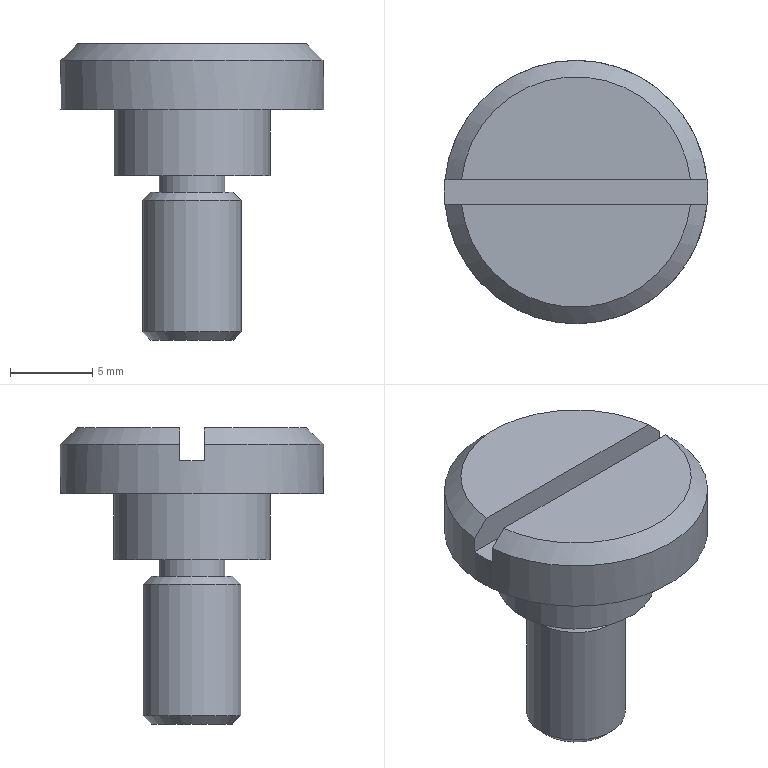Component | NX | DRILL_BUSHING_SCREW_3 | 1 solid | 17 faces | box 16 x 16 x 18 mm | volume 1280 mm3 | plane 9 | cylinder 4 | cone 4 | commonest cylinder face diameters 6 x1 4 x1 9.5 x1 16 x1
STEP:
#1=CARTESIAN_POINT('',(0.,0.,0.));
#2=DIRECTION('',(0.,0.,1.));
#3=DIRECTION('',(1.,0.,0.));
#4=AXIS2_PLACEMENT_3D('',#1,#2,#3);
#5=CARTESIAN_POINT('',(329.141,43.75,118.));
#6=VERTEX_POINT('',#5);
#7=CARTESIAN_POINT('',(343.061,43.75,118.));
#8=VERTEX_POINT('',#7);
#9=CARTESIAN_POINT('',(322.351,43.75,118.));
#10=DIRECTION('',(1.,0.,0.));
#11=VECTOR('',#10,1.);
#12=LINE('',#9,#11);
#13=CARTESIAN_POINT('',(336.101,44.5,118.));
#14=DIRECTION('',(0.,0.,1.));
#15=DIRECTION('',(1.,0.,0.));
#16=AXIS2_PLACEMENT_3D('',#13,#14,#15);
#17=PLANE('',#16);
#18=CARTESIAN_POINT('',(-13.75,-0.75));
#19=DIRECTION('',(1.,0.));
#20=VECTOR('',#19,1.);
#21=LINE('',#18,#20);
#22=(GEOMETRIC_REPRESENTATION_CONTEXT(2)PARAMETRIC_REPRESENTATION_CONTEXT()REPRESENTATION_CONTEXT('',''));
#23=DEFINITIONAL_REPRESENTATION('',(#21),#22);
#24=PCURVE('',#17,#23);
#25=CARTESIAN_POINT('',(322.351,43.75,116.));
#26=DIRECTION('',(0.,-1.,0.));
#27=DIRECTION('',(0.,0.,-1.));
#28=AXIS2_PLACEMENT_3D('',#25,#26,#27);
#29=PLANE('',#28);
#30=CARTESIAN_POINT('',(-2.,0.));
#31=DIRECTION('',(0.,1.));
#32=VECTOR('',#31,1.);
#33=LINE('',#30,#32);
#34=(GEOMETRIC_REPRESENTATION_CONTEXT(2)PARAMETRIC_REPRESENTATION_CONTEXT()REPRESENTATION_CONTEXT('',''));
#35=DEFINITIONAL_REPRESENTATION('',(#33),#34);
#36=PCURVE('',#29,#35);
#37=SURFACE_CURVE('',#12,(#24,#36),.PCURVE_S1.);
#38=EDGE_CURVE('',#6,#8,#37,.T.);
#39=ORIENTED_EDGE('',*,*,#38,.F.);
#40=CARTESIAN_POINT('',(336.101,44.5,118.));
#41=DIRECTION('',(0.,0.,1.));
#42=DIRECTION('',(1.,0.,0.));
#43=AXIS2_PLACEMENT_3D('',#40,#41,#42);
#44=CIRCLE('',#43,7.);
#45=CARTESIAN_POINT('',(0.,0.));
#46=DIRECTION('',(1.,0.));
#47=AXIS2_PLACEMENT_2D('',#45,#46);
#48=CIRCLE('',#47,7.);
#49=(GEOMETRIC_REPRESENTATION_CONTEXT(2)PARAMETRIC_REPRESENTATION_CONTEXT()REPRESENTATION_CONTEXT('',''));
#50=DEFINITIONAL_REPRESENTATION('',(#48),#49);
#51=PCURVE('',#17,#50);
#52=CARTESIAN_POINT('',(336.101,44.5,117.));
#53=DIRECTION('',(0.,0.,-1.));
#54=DIRECTION('',(-1.,0.,0.));
#55=AXIS2_PLACEMENT_3D('',#52,#53,#54);
#56=CONICAL_SURFACE('',#55,8.,0.7854);
#57=CARTESIAN_POINT('',(9.425,-1.));
#58=DIRECTION('',(-1.,-0.));
#59=VECTOR('',#58,1.);
#60=LINE('',#57,#59);
#61=(GEOMETRIC_REPRESENTATION_CONTEXT(2)PARAMETRIC_REPRESENTATION_CONTEXT()REPRESENTATION_CONTEXT('',''));
#62=DEFINITIONAL_REPRESENTATION('',(#60),#61);
#63=PCURVE('',#56,#62);
#64=SURFACE_CURVE('',#44,(#51,#63),.PCURVE_S1.);
#65=EDGE_CURVE('',#6,#8,#64,.T.);
#66=ORIENTED_EDGE('',*,*,#65,.T.);
#67=EDGE_LOOP('',(#39,#66));
#68=FACE_BOUND('',#67,.T.);
#69=ADVANCED_FACE('',(#68),#17,.T.);
#70=CARTESIAN_POINT('',(338.601,44.5,109.));
#71=VERTEX_POINT('',#70);
#72=CARTESIAN_POINT('',(336.101,44.5,109.));
#73=DIRECTION('',(0.,0.,1.));
#74=DIRECTION('',(1.,0.,0.));
#75=AXIS2_PLACEMENT_3D('',#72,#73,#74);
#76=CIRCLE('',#75,2.5);
#77=CARTESIAN_POINT('',(336.101,44.5,109.));
#78=DIRECTION('',(0.,0.,1.));
#79=DIRECTION('',(1.,0.,0.));
#80=AXIS2_PLACEMENT_3D('',#77,#78,#79);
#81=PLANE('',#80);
#82=CARTESIAN_POINT('',(0.,0.));
#83=DIRECTION('',(1.,0.));
#84=AXIS2_PLACEMENT_2D('',#82,#83);
#85=CIRCLE('',#84,2.5);
#86=(GEOMETRIC_REPRESENTATION_CONTEXT(2)PARAMETRIC_REPRESENTATION_CONTEXT()REPRESENTATION_CONTEXT('',''));
#87=DEFINITIONAL_REPRESENTATION('',(#85),#86);
#88=PCURVE('',#81,#87);
#89=CARTESIAN_POINT('',(336.101,44.5,108.5));
#90=DIRECTION('',(0.,0.,-1.));
#91=DIRECTION('',(-1.,0.,0.));
#92=AXIS2_PLACEMENT_3D('',#89,#90,#91);
#93=CONICAL_SURFACE('',#92,3.,0.7854);
#94=CARTESIAN_POINT('',(9.425,-0.5));
#95=DIRECTION('',(-1.,0.));
#96=VECTOR('',#95,1.);
#97=LINE('',#94,#96);
#98=(GEOMETRIC_REPRESENTATION_CONTEXT(2)PARAMETRIC_REPRESENTATION_CONTEXT()REPRESENTATION_CONTEXT('',''));
#99=DEFINITIONAL_REPRESENTATION('',(#97),#98);
#100=PCURVE('',#93,#99);
#101=SURFACE_CURVE('',#76,(#88,#100),.PCURVE_S1.);
#102=EDGE_CURVE('',#71,#71,#101,.T.);
#103=ORIENTED_EDGE('',*,*,#102,.T.);
#104=EDGE_LOOP('',(#103));
#105=FACE_BOUND('',#104,.T.);
#106=CARTESIAN_POINT('',(338.101,44.5,109.));
#107=VERTEX_POINT('',#106);
#108=CARTESIAN_POINT('',(336.101,44.5,109.));
#109=DIRECTION('',(0.,0.,1.));
#110=DIRECTION('',(1.,0.,0.));
#111=AXIS2_PLACEMENT_3D('',#108,#109,#110);
#112=CIRCLE('',#111,2.);
#113=CARTESIAN_POINT('',(0.,0.));
#114=DIRECTION('',(1.,0.));
#115=AXIS2_PLACEMENT_2D('',#113,#114);
#116=CIRCLE('',#115,2.);
#117=(GEOMETRIC_REPRESENTATION_CONTEXT(2)PARAMETRIC_REPRESENTATION_CONTEXT()REPRESENTATION_CONTEXT('',''));
#118=DEFINITIONAL_REPRESENTATION('',(#116),#117);
#119=PCURVE('',#81,#118);
#120=CARTESIAN_POINT('',(336.101,44.5,109.));
#121=DIRECTION('',(0.,0.,1.));
#122=DIRECTION('',(1.,0.,0.));
#123=AXIS2_PLACEMENT_3D('',#120,#121,#122);
#124=CYLINDRICAL_SURFACE('',#123,2.);
#125=CARTESIAN_POINT('',(0.,0.));
#126=DIRECTION('',(1.,0.));
#127=VECTOR('',#126,1.);
#128=LINE('',#125,#127);
#129=(GEOMETRIC_REPRESENTATION_CONTEXT(2)PARAMETRIC_REPRESENTATION_CONTEXT()REPRESENTATION_CONTEXT('',''));
#130=DEFINITIONAL_REPRESENTATION('',(#128),#129);
#131=PCURVE('',#124,#130);
#132=SURFACE_CURVE('',#112,(#119,#131),.PCURVE_S1.);
#133=EDGE_CURVE('',#107,#107,#132,.T.);
#134=ORIENTED_EDGE('',*,*,#133,.F.);
#135=EDGE_LOOP('',(#134));
#136=FACE_BOUND('',#135,.T.);
#137=ADVANCED_FACE('',(#105,#136),#81,.T.);
#138=CARTESIAN_POINT('',(333.601,44.5,100.));
#139=VERTEX_POINT('',#138);
#140=CARTESIAN_POINT('',(336.101,44.5,100.));
#141=DIRECTION('',(0.,0.,-1.));
#142=DIRECTION('',(-1.,0.,0.));
#143=AXIS2_PLACEMENT_3D('',#140,#141,#142);
#144=CIRCLE('',#143,2.5);
#145=CARTESIAN_POINT('',(336.101,44.5,100.));
#146=DIRECTION('',(0.,0.,-1.));
#147=DIRECTION('',(-1.,0.,0.));
#148=AXIS2_PLACEMENT_3D('',#145,#146,#147);
#149=PLANE('',#148);
#150=CARTESIAN_POINT('',(0.,0.));
#151=DIRECTION('',(1.,0.));
#152=AXIS2_PLACEMENT_2D('',#150,#151);
#153=CIRCLE('',#152,2.5);
#154=(GEOMETRIC_REPRESENTATION_CONTEXT(2)PARAMETRIC_REPRESENTATION_CONTEXT()REPRESENTATION_CONTEXT('',''));
#155=DEFINITIONAL_REPRESENTATION('',(#153),#154);
#156=PCURVE('',#149,#155);
#157=CARTESIAN_POINT('',(336.101,44.5,100.5));
#158=DIRECTION('',(0.,0.,1.));
#159=DIRECTION('',(1.,0.,0.));
#160=AXIS2_PLACEMENT_3D('',#157,#158,#159);
#161=CONICAL_SURFACE('',#160,3.,0.7854);
#162=CARTESIAN_POINT('',(9.425,-0.5));
#163=DIRECTION('',(-1.,0.));
#164=VECTOR('',#163,1.);
#165=LINE('',#162,#164);
#166=(GEOMETRIC_REPRESENTATION_CONTEXT(2)PARAMETRIC_REPRESENTATION_CONTEXT()REPRESENTATION_CONTEXT('',''));
#167=DEFINITIONAL_REPRESENTATION('',(#165),#166);
#168=PCURVE('',#161,#167);
#169=SURFACE_CURVE('',#144,(#156,#168),.PCURVE_S1.);
#170=EDGE_CURVE('',#139,#139,#169,.T.);
#171=ORIENTED_EDGE('',*,*,#170,.T.);
#172=EDGE_LOOP('',(#171));
#173=FACE_BOUND('',#172,.T.);
#174=ADVANCED_FACE('',(#173),#149,.T.);
#175=CARTESIAN_POINT('',(333.101,44.5,100.5));
#176=VERTEX_POINT('',#175);
#177=CARTESIAN_POINT('',(339.101,44.5,100.5));
#178=VERTEX_POINT('',#177);
#179=CARTESIAN_POINT('',(336.101,44.5,100.5));
#180=DIRECTION('',(0.,0.,1.));
#181=DIRECTION('',(-1.,0.,0.));
#182=AXIS2_PLACEMENT_3D('',#179,#180,#181);
#183=CIRCLE('',#182,3.);
#184=CARTESIAN_POINT('',(336.101,44.5,100.));
#185=DIRECTION('',(0.,0.,1.));
#186=DIRECTION('',(1.,0.,0.));
#187=AXIS2_PLACEMENT_3D('',#184,#185,#186);
#188=CYLINDRICAL_SURFACE('',#187,3.);
#189=CARTESIAN_POINT('',(3.142,0.5));
#190=DIRECTION('',(1.,0.));
#191=VECTOR('',#190,1.);
#192=LINE('',#189,#191);
#193=(GEOMETRIC_REPRESENTATION_CONTEXT(2)PARAMETRIC_REPRESENTATION_CONTEXT()REPRESENTATION_CONTEXT('',''));
#194=DEFINITIONAL_REPRESENTATION('',(#192),#193);
#195=PCURVE('',#188,#194);
#196=CARTESIAN_POINT('',(3.142,0.));
#197=DIRECTION('',(1.,0.));
#198=VECTOR('',#197,1.);
#199=LINE('',#196,#198);
#200=(GEOMETRIC_REPRESENTATION_CONTEXT(2)PARAMETRIC_REPRESENTATION_CONTEXT()REPRESENTATION_CONTEXT('',''));
#201=DEFINITIONAL_REPRESENTATION('',(#199),#200);
#202=PCURVE('',#161,#201);
#203=SURFACE_CURVE('',#183,(#195,#202),.PCURVE_S1.);
#204=EDGE_CURVE('',#176,#178,#203,.T.);
#205=ORIENTED_EDGE('',*,*,#204,.T.);
#206=CARTESIAN_POINT('',(339.101,44.5,108.5));
#207=VERTEX_POINT('',#206);
#208=CARTESIAN_POINT('',(339.101,44.5,100.5));
#209=CARTESIAN_POINT('',(339.101,44.5,108.5));
#210=B_SPLINE_CURVE_WITH_KNOTS('',1,(#208,#209),.UNSPECIFIED.,.F.,.F.,(2,2),(0.5,8.5),.PIECEWISE_BEZIER_KNOTS.);
#211=CARTESIAN_POINT('',(6.283,0.));
#212=DIRECTION('',(0.,1.));
#213=VECTOR('',#212,1.);
#214=LINE('',#211,#213);
#215=(GEOMETRIC_REPRESENTATION_CONTEXT(2)PARAMETRIC_REPRESENTATION_CONTEXT()REPRESENTATION_CONTEXT('',''));
#216=DEFINITIONAL_REPRESENTATION('',(#214),#215);
#217=PCURVE('',#188,#216);
#218=CARTESIAN_POINT('',(0.,0.));
#219=DIRECTION('',(0.,1.));
#220=VECTOR('',#219,1.);
#221=LINE('',#218,#220);
#222=(GEOMETRIC_REPRESENTATION_CONTEXT(2)PARAMETRIC_REPRESENTATION_CONTEXT()REPRESENTATION_CONTEXT('',''));
#223=DEFINITIONAL_REPRESENTATION('',(#221),#222);
#224=PCURVE('',#188,#223);
#225=SEAM_CURVE('',#210,(#217,#224),.PCURVE_S1.);
#226=EDGE_CURVE('',#178,#207,#225,.T.);
#227=ORIENTED_EDGE('',*,*,#226,.T.);
#228=CARTESIAN_POINT('',(336.101,44.5,108.5));
#229=DIRECTION('',(0.,0.,-1.));
#230=DIRECTION('',(1.,0.,0.));
#231=AXIS2_PLACEMENT_3D('',#228,#229,#230);
#232=CIRCLE('',#231,3.);
#233=CARTESIAN_POINT('',(6.283,8.5));
#234=DIRECTION('',(-1.,0.));
#235=VECTOR('',#234,1.);
#236=LINE('',#233,#235);
#237=(GEOMETRIC_REPRESENTATION_CONTEXT(2)PARAMETRIC_REPRESENTATION_CONTEXT()REPRESENTATION_CONTEXT('',''));
#238=DEFINITIONAL_REPRESENTATION('',(#236),#237);
#239=PCURVE('',#188,#238);
#240=CARTESIAN_POINT('',(3.142,0.));
#241=DIRECTION('',(1.,0.));
#242=VECTOR('',#241,1.);
#243=LINE('',#240,#242);
#244=(GEOMETRIC_REPRESENTATION_CONTEXT(2)PARAMETRIC_REPRESENTATION_CONTEXT()REPRESENTATION_CONTEXT('',''));
#245=DEFINITIONAL_REPRESENTATION('',(#243),#244);
#246=PCURVE('',#93,#245);
#247=SURFACE_CURVE('',#232,(#239,#246),.PCURVE_S1.);
#248=EDGE_CURVE('',#207,#207,#247,.T.);
#249=ORIENTED_EDGE('',*,*,#248,.T.);
#250=ORIENTED_EDGE('',*,*,#226,.F.);
#251=CARTESIAN_POINT('',(336.101,44.5,100.5));
#252=DIRECTION('',(0.,0.,1.));
#253=DIRECTION('',(-1.,0.,0.));
#254=AXIS2_PLACEMENT_3D('',#251,#252,#253);
#255=CIRCLE('',#254,3.);
#256=CARTESIAN_POINT('',(-3.142,0.5));
#257=DIRECTION('',(1.,0.));
#258=VECTOR('',#257,1.);
#259=LINE('',#256,#258);
#260=(GEOMETRIC_REPRESENTATION_CONTEXT(2)PARAMETRIC_REPRESENTATION_CONTEXT()REPRESENTATION_CONTEXT('',''));
#261=DEFINITIONAL_REPRESENTATION('',(#259),#260);
#262=PCURVE('',#188,#261);
#263=CARTESIAN_POINT('',(3.142,0.));
#264=DIRECTION('',(1.,0.));
#265=VECTOR('',#264,1.);
#266=LINE('',#263,#265);
#267=(GEOMETRIC_REPRESENTATION_CONTEXT(2)PARAMETRIC_REPRESENTATION_CONTEXT()REPRESENTATION_CONTEXT('',''));
#268=DEFINITIONAL_REPRESENTATION('',(#266),#267);
#269=PCURVE('',#161,#268);
#270=SURFACE_CURVE('',#255,(#262,#269),.PCURVE_S1.);
#271=EDGE_CURVE('',#178,#176,#270,.T.);
#272=ORIENTED_EDGE('',*,*,#271,.T.);
#273=EDGE_LOOP('',(#205,#227,#249,#250,#272));
#274=FACE_BOUND('',#273,.T.);
#275=ADVANCED_FACE('',(#274),#188,.T.);
#276=CARTESIAN_POINT('',(338.101,44.5,110.));
#277=VERTEX_POINT('',#276);
#278=CARTESIAN_POINT('',(336.101,44.5,110.));
#279=DIRECTION('',(0.,0.,-1.));
#280=DIRECTION('',(1.,0.,0.));
#281=AXIS2_PLACEMENT_3D('',#278,#279,#280);
#282=CIRCLE('',#281,2.);
#283=CARTESIAN_POINT('',(6.283,1.));
#284=DIRECTION('',(-1.,0.));
#285=VECTOR('',#284,1.);
#286=LINE('',#283,#285);
#287=(GEOMETRIC_REPRESENTATION_CONTEXT(2)PARAMETRIC_REPRESENTATION_CONTEXT()REPRESENTATION_CONTEXT('',''));
#288=DEFINITIONAL_REPRESENTATION('',(#286),#287);
#289=PCURVE('',#124,#288);
#290=CARTESIAN_POINT('',(336.101,44.5,110.));
#291=DIRECTION('',(0.,0.,-1.));
#292=DIRECTION('',(-1.,0.,0.));
#293=AXIS2_PLACEMENT_3D('',#290,#291,#292);
#294=PLANE('',#293);
#295=CARTESIAN_POINT('',(0.,0.));
#296=DIRECTION('',(-1.,0.));
#297=AXIS2_PLACEMENT_2D('',#295,#296);
#298=CIRCLE('',#297,2.);
#299=(GEOMETRIC_REPRESENTATION_CONTEXT(2)PARAMETRIC_REPRESENTATION_CONTEXT()REPRESENTATION_CONTEXT('',''));
#300=DEFINITIONAL_REPRESENTATION('',(#298),#299);
#301=PCURVE('',#294,#300);
#302=SURFACE_CURVE('',#282,(#289,#301),.PCURVE_S1.);
#303=EDGE_CURVE('',#277,#277,#302,.T.);
#304=ORIENTED_EDGE('',*,*,#303,.T.);
#305=CARTESIAN_POINT('',(338.101,44.5,109.));
#306=CARTESIAN_POINT('',(338.101,44.5,110.));
#307=B_SPLINE_CURVE_WITH_KNOTS('',1,(#305,#306),.UNSPECIFIED.,.F.,.F.,(2,2),(0.,1.),.PIECEWISE_BEZIER_KNOTS.);
#308=CARTESIAN_POINT('',(0.,0.));
#309=DIRECTION('',(0.,1.));
#310=VECTOR('',#309,1.);
#311=LINE('',#308,#310);
#312=(GEOMETRIC_REPRESENTATION_CONTEXT(2)PARAMETRIC_REPRESENTATION_CONTEXT()REPRESENTATION_CONTEXT('',''));
#313=DEFINITIONAL_REPRESENTATION('',(#311),#312);
#314=PCURVE('',#124,#313);
#315=CARTESIAN_POINT('',(6.283,0.));
#316=DIRECTION('',(0.,1.));
#317=VECTOR('',#316,1.);
#318=LINE('',#315,#317);
#319=(GEOMETRIC_REPRESENTATION_CONTEXT(2)PARAMETRIC_REPRESENTATION_CONTEXT()REPRESENTATION_CONTEXT('',''));
#320=DEFINITIONAL_REPRESENTATION('',(#318),#319);
#321=PCURVE('',#124,#320);
#322=SEAM_CURVE('',#307,(#314,#321),.PCURVE_S1.);
#323=EDGE_CURVE('',#107,#277,#322,.T.);
#324=ORIENTED_EDGE('',*,*,#323,.F.);
#325=ORIENTED_EDGE('',*,*,#133,.T.);
#326=ORIENTED_EDGE('',*,*,#323,.T.);
#327=EDGE_LOOP('',(#304,#324,#325,#326));
#328=FACE_BOUND('',#327,.T.);
#329=ADVANCED_FACE('',(#328),#124,.T.);
#330=ORIENTED_EDGE('',*,*,#303,.F.);
#331=EDGE_LOOP('',(#330));
#332=FACE_BOUND('',#331,.T.);
#333=CARTESIAN_POINT('',(340.851,44.5,110.));
#334=VERTEX_POINT('',#333);
#335=CARTESIAN_POINT('',(336.101,44.5,110.));
#336=DIRECTION('',(0.,0.,1.));
#337=DIRECTION('',(1.,0.,0.));
#338=AXIS2_PLACEMENT_3D('',#335,#336,#337);
#339=CIRCLE('',#338,4.75);
#340=CARTESIAN_POINT('',(-4.75,0.));
#341=CARTESIAN_POINT('',(-4.75,8.227));
#342=CARTESIAN_POINT('',(2.375,4.114));
#343=CARTESIAN_POINT('',(9.5,0.));
#344=CARTESIAN_POINT('',(2.375,-4.114));
#345=CARTESIAN_POINT('',(-4.75,-8.227));
#346=CARTESIAN_POINT('',(-4.75,0.));
#347=(BOUNDED_CURVE()B_SPLINE_CURVE(2,(#340,#341,#342,#343,#344,#345,#346),.UNSPECIFIED.,.T.,.F.)B_SPLINE_CURVE_WITH_KNOTS((1,2,2,2,2,1),(-2.094,0.,2.094,4.189,6.283,8.378),.UNSPECIFIED.)CURVE()GEOMETRIC_REPRESENTATION_ITEM()RATIONAL_B_SPLINE_CURVE((1.,0.5,1.,0.5,1.,0.5,1.))REPRESENTATION_ITEM(''));
#348=(GEOMETRIC_REPRESENTATION_CONTEXT(2)PARAMETRIC_REPRESENTATION_CONTEXT()REPRESENTATION_CONTEXT('',''));
#349=DEFINITIONAL_REPRESENTATION('',(#347),#348);
#350=PCURVE('',#294,#349);
#351=CARTESIAN_POINT('',(336.101,44.5,110.));
#352=DIRECTION('',(0.,0.,1.));
#353=DIRECTION('',(1.,0.,0.));
#354=AXIS2_PLACEMENT_3D('',#351,#352,#353);
#355=CYLINDRICAL_SURFACE('',#354,4.75);
#356=CARTESIAN_POINT('',(0.,0.));
#357=DIRECTION('',(1.,0.));
#358=VECTOR('',#357,1.);
#359=LINE('',#356,#358);
#360=(GEOMETRIC_REPRESENTATION_CONTEXT(2)PARAMETRIC_REPRESENTATION_CONTEXT()REPRESENTATION_CONTEXT('',''));
#361=DEFINITIONAL_REPRESENTATION('',(#359),#360);
#362=PCURVE('',#355,#361);
#363=SURFACE_CURVE('',#339,(#350,#362),.PCURVE_S1.);
#364=EDGE_CURVE('',#334,#334,#363,.T.);
#365=ORIENTED_EDGE('',*,*,#364,.F.);
#366=EDGE_LOOP('',(#365));
#367=FACE_BOUND('',#366,.T.);
#368=ADVANCED_FACE('',(#332,#367),#294,.T.);
#369=CARTESIAN_POINT('',(340.851,44.5,114.));
#370=VERTEX_POINT('',#369);
#371=CARTESIAN_POINT('',(336.101,44.5,114.));
#372=DIRECTION('',(0.,0.,-1.));
#373=DIRECTION('',(1.,0.,0.));
#374=AXIS2_PLACEMENT_3D('',#371,#372,#373);
#375=CIRCLE('',#374,4.75);
#376=CARTESIAN_POINT('',(6.283,4.));
#377=DIRECTION('',(-1.,0.));
#378=VECTOR('',#377,1.);
#379=LINE('',#376,#378);
#380=(GEOMETRIC_REPRESENTATION_CONTEXT(2)PARAMETRIC_REPRESENTATION_CONTEXT()REPRESENTATION_CONTEXT('',''));
#381=DEFINITIONAL_REPRESENTATION('',(#379),#380);
#382=PCURVE('',#355,#381);
#383=CARTESIAN_POINT('',(336.101,44.5,114.));
#384=DIRECTION('',(0.,0.,-1.));
#385=DIRECTION('',(-1.,0.,0.));
#386=AXIS2_PLACEMENT_3D('',#383,#384,#385);
#387=PLANE('',#386);
#388=CARTESIAN_POINT('',(0.,0.));
#389=DIRECTION('',(-1.,0.));
#390=AXIS2_PLACEMENT_2D('',#388,#389);
#391=CIRCLE('',#390,4.75);
#392=(GEOMETRIC_REPRESENTATION_CONTEXT(2)PARAMETRIC_REPRESENTATION_CONTEXT()REPRESENTATION_CONTEXT('',''));
#393=DEFINITIONAL_REPRESENTATION('',(#391),#392);
#394=PCURVE('',#387,#393);
#395=SURFACE_CURVE('',#375,(#382,#394),.PCURVE_S1.);
#396=EDGE_CURVE('',#370,#370,#395,.T.);
#397=ORIENTED_EDGE('',*,*,#396,.T.);
#398=CARTESIAN_POINT('',(340.851,44.5,110.));
#399=CARTESIAN_POINT('',(340.851,44.5,114.));
#400=B_SPLINE_CURVE_WITH_KNOTS('',1,(#398,#399),.UNSPECIFIED.,.F.,.F.,(2,2),(0.,4.),.PIECEWISE_BEZIER_KNOTS.);
#401=CARTESIAN_POINT('',(0.,0.));
#402=DIRECTION('',(0.,1.));
#403=VECTOR('',#402,1.);
#404=LINE('',#401,#403);
#405=(GEOMETRIC_REPRESENTATION_CONTEXT(2)PARAMETRIC_REPRESENTATION_CONTEXT()REPRESENTATION_CONTEXT('',''));
#406=DEFINITIONAL_REPRESENTATION('',(#404),#405);
#407=PCURVE('',#355,#406);
#408=CARTESIAN_POINT('',(6.283,0.));
#409=DIRECTION('',(0.,1.));
#410=VECTOR('',#409,1.);
#411=LINE('',#408,#410);
#412=(GEOMETRIC_REPRESENTATION_CONTEXT(2)PARAMETRIC_REPRESENTATION_CONTEXT()REPRESENTATION_CONTEXT('',''));
#413=DEFINITIONAL_REPRESENTATION('',(#411),#412);
#414=PCURVE('',#355,#413);
#415=SEAM_CURVE('',#400,(#407,#414),.PCURVE_S1.);
#416=EDGE_CURVE('',#334,#370,#415,.T.);
#417=ORIENTED_EDGE('',*,*,#416,.F.);
#418=ORIENTED_EDGE('',*,*,#364,.T.);
#419=ORIENTED_EDGE('',*,*,#416,.T.);
#420=EDGE_LOOP('',(#397,#417,#418,#419));
#421=FACE_BOUND('',#420,.T.);
#422=ADVANCED_FACE('',(#421),#355,.T.);
#423=CARTESIAN_POINT('',(343.061,45.25,118.));
#424=VERTEX_POINT('',#423);
#425=CARTESIAN_POINT('',(329.141,45.25,118.));
#426=VERTEX_POINT('',#425);
#427=CARTESIAN_POINT('',(349.851,45.25,118.));
#428=DIRECTION('',(-1.,0.,0.));
#429=VECTOR('',#428,1.);
#430=LINE('',#427,#429);
#431=CARTESIAN_POINT('',(336.101,44.5,118.));
#432=DIRECTION('',(0.,0.,1.));
#433=DIRECTION('',(1.,0.,0.));
#434=AXIS2_PLACEMENT_3D('',#431,#432,#433);
#435=PLANE('',#434);
#436=CARTESIAN_POINT('',(13.75,0.75));
#437=DIRECTION('',(-1.,0.));
#438=VECTOR('',#437,1.);
#439=LINE('',#436,#438);
#440=(GEOMETRIC_REPRESENTATION_CONTEXT(2)PARAMETRIC_REPRESENTATION_CONTEXT()REPRESENTATION_CONTEXT('',''));
#441=DEFINITIONAL_REPRESENTATION('',(#439),#440);
#442=PCURVE('',#435,#441);
#443=CARTESIAN_POINT('',(349.851,45.25,116.));
#444=DIRECTION('',(0.,1.,0.));
#445=DIRECTION('',(0.,0.,1.));
#446=AXIS2_PLACEMENT_3D('',#443,#444,#445);
#447=PLANE('',#446);
#448=CARTESIAN_POINT('',(2.,0.));
#449=DIRECTION('',(0.,-1.));
#450=VECTOR('',#449,1.);
#451=LINE('',#448,#450);
#452=(GEOMETRIC_REPRESENTATION_CONTEXT(2)PARAMETRIC_REPRESENTATION_CONTEXT()REPRESENTATION_CONTEXT('',''));
#453=DEFINITIONAL_REPRESENTATION('',(#451),#452);
#454=PCURVE('',#447,#453);
#455=SURFACE_CURVE('',#430,(#442,#454),.PCURVE_S1.);
#456=EDGE_CURVE('',#424,#426,#455,.T.);
#457=ORIENTED_EDGE('',*,*,#456,.F.);
#458=CARTESIAN_POINT('',(336.101,44.5,118.));
#459=DIRECTION('',(0.,0.,1.));
#460=DIRECTION('',(1.,0.,0.));
#461=AXIS2_PLACEMENT_3D('',#458,#459,#460);
#462=CIRCLE('',#461,7.);
#463=CARTESIAN_POINT('',(0.,0.));
#464=DIRECTION('',(1.,0.));
#465=AXIS2_PLACEMENT_2D('',#463,#464);
#466=CIRCLE('',#465,7.);
#467=(GEOMETRIC_REPRESENTATION_CONTEXT(2)PARAMETRIC_REPRESENTATION_CONTEXT()REPRESENTATION_CONTEXT('',''));
#468=DEFINITIONAL_REPRESENTATION('',(#466),#467);
#469=PCURVE('',#435,#468);
#470=CARTESIAN_POINT('',(336.101,44.5,117.));
#471=DIRECTION('',(0.,0.,-1.));
#472=DIRECTION('',(-1.,0.,0.));
#473=AXIS2_PLACEMENT_3D('',#470,#471,#472);
#474=CONICAL_SURFACE('',#473,8.,0.7854);
#475=CARTESIAN_POINT('',(3.142,-1.));
#476=DIRECTION('',(-1.,0.));
#477=VECTOR('',#476,1.);
#478=LINE('',#475,#477);
#479=(GEOMETRIC_REPRESENTATION_CONTEXT(2)PARAMETRIC_REPRESENTATION_CONTEXT()REPRESENTATION_CONTEXT('',''));
#480=DEFINITIONAL_REPRESENTATION('',(#478),#479);
#481=PCURVE('',#474,#480);
#482=SURFACE_CURVE('',#462,(#469,#481),.PCURVE_S1.);
#483=EDGE_CURVE('',#424,#426,#482,.T.);
#484=ORIENTED_EDGE('',*,*,#483,.T.);
#485=EDGE_LOOP('',(#457,#484));
#486=FACE_BOUND('',#485,.T.);
#487=ADVANCED_FACE('',(#486),#435,.T.);
#488=ORIENTED_EDGE('',*,*,#396,.F.);
#489=EDGE_LOOP('',(#488));
#490=FACE_BOUND('',#489,.T.);
#491=CARTESIAN_POINT('',(344.101,44.5,114.));
#492=VERTEX_POINT('',#491);
#493=CARTESIAN_POINT('',(336.101,44.5,114.));
#494=DIRECTION('',(0.,0.,1.));
#495=DIRECTION('',(1.,0.,0.));
#496=AXIS2_PLACEMENT_3D('',#493,#494,#495);
#497=CIRCLE('',#496,8.);
#498=CARTESIAN_POINT('',(-8.,0.));
#499=CARTESIAN_POINT('',(-8.,13.856));
#500=CARTESIAN_POINT('',(4.,6.928));
#501=CARTESIAN_POINT('',(16.,0.));
#502=CARTESIAN_POINT('',(4.,-6.928));
#503=CARTESIAN_POINT('',(-8.,-13.856));
#504=CARTESIAN_POINT('',(-8.,0.));
#505=(BOUNDED_CURVE()B_SPLINE_CURVE(2,(#498,#499,#500,#501,#502,#503,#504),.UNSPECIFIED.,.T.,.F.)B_SPLINE_CURVE_WITH_KNOTS((1,2,2,2,2,1),(-2.094,0.,2.094,4.189,6.283,8.378),.UNSPECIFIED.)CURVE()GEOMETRIC_REPRESENTATION_ITEM()RATIONAL_B_SPLINE_CURVE((1.,0.5,1.,0.5,1.,0.5,1.))REPRESENTATION_ITEM(''));
#506=(GEOMETRIC_REPRESENTATION_CONTEXT(2)PARAMETRIC_REPRESENTATION_CONTEXT()REPRESENTATION_CONTEXT('',''));
#507=DEFINITIONAL_REPRESENTATION('',(#505),#506);
#508=PCURVE('',#387,#507);
#509=CARTESIAN_POINT('',(336.101,44.5,114.));
#510=DIRECTION('',(0.,0.,1.));
#511=DIRECTION('',(1.,0.,0.));
#512=AXIS2_PLACEMENT_3D('',#509,#510,#511);
#513=CYLINDRICAL_SURFACE('',#512,8.);
#514=CARTESIAN_POINT('',(0.,0.));
#515=DIRECTION('',(1.,0.));
#516=VECTOR('',#515,1.);
#517=LINE('',#514,#516);
#518=(GEOMETRIC_REPRESENTATION_CONTEXT(2)PARAMETRIC_REPRESENTATION_CONTEXT()REPRESENTATION_CONTEXT('',''));
#519=DEFINITIONAL_REPRESENTATION('',(#517),#518);
#520=PCURVE('',#513,#519);
#521=SURFACE_CURVE('',#497,(#508,#520),.PCURVE_S1.);
#522=EDGE_CURVE('',#492,#492,#521,.T.);
#523=ORIENTED_EDGE('',*,*,#522,.F.);
#524=EDGE_LOOP('',(#523));
#525=FACE_BOUND('',#524,.T.);
#526=ADVANCED_FACE('',(#490,#525),#387,.T.);
#527=CARTESIAN_POINT('',(328.136,45.25,117.));
#528=VERTEX_POINT('',#527);
#529=CARTESIAN_POINT('',(328.136,45.25,116.));
#530=VERTEX_POINT('',#529);
#531=CARTESIAN_POINT('',(328.136,45.25,114.));
#532=DIRECTION('',(0.,0.,-1.));
#533=VECTOR('',#532,1.);
#534=LINE('',#531,#533);
#535=CARTESIAN_POINT('',(3.048,0.));
#536=DIRECTION('',(0.,-1.));
#537=VECTOR('',#536,1.);
#538=LINE('',#535,#537);
#539=(GEOMETRIC_REPRESENTATION_CONTEXT(2)PARAMETRIC_REPRESENTATION_CONTEXT()REPRESENTATION_CONTEXT('',''));
#540=DEFINITIONAL_REPRESENTATION('',(#538),#539);
#541=PCURVE('',#513,#540);
#542=CARTESIAN_POINT('',(-2.,-21.715));
#543=DIRECTION('',(-1.,0.));
#544=VECTOR('',#543,1.);
#545=LINE('',#542,#544);
#546=(GEOMETRIC_REPRESENTATION_CONTEXT(2)PARAMETRIC_REPRESENTATION_CONTEXT()REPRESENTATION_CONTEXT('',''));
#547=DEFINITIONAL_REPRESENTATION('',(#545),#546);
#548=PCURVE('',#447,#547);
#549=SURFACE_CURVE('',#534,(#541,#548),.PCURVE_S1.);
#550=EDGE_CURVE('',#528,#530,#549,.T.);
#551=ORIENTED_EDGE('',*,*,#550,.F.);
#552=CARTESIAN_POINT('',(344.066,45.25,117.));
#553=VERTEX_POINT('',#552);
#554=CARTESIAN_POINT('',(336.101,44.5,117.));
#555=DIRECTION('',(0.,0.,-1.));
#556=DIRECTION('',(1.,0.,0.));
#557=AXIS2_PLACEMENT_3D('',#554,#555,#556);
#558=CIRCLE('',#557,8.);
#559=CARTESIAN_POINT('',(6.283,3.));
#560=DIRECTION('',(-1.,0.));
#561=VECTOR('',#560,1.);
#562=LINE('',#559,#561);
#563=(GEOMETRIC_REPRESENTATION_CONTEXT(2)PARAMETRIC_REPRESENTATION_CONTEXT()REPRESENTATION_CONTEXT('',''));
#564=DEFINITIONAL_REPRESENTATION('',(#562),#563);
#565=PCURVE('',#513,#564);
#566=CARTESIAN_POINT('',(-3.142,0.));
#567=DIRECTION('',(1.,0.));
#568=VECTOR('',#567,1.);
#569=LINE('',#566,#568);
#570=(GEOMETRIC_REPRESENTATION_CONTEXT(2)PARAMETRIC_REPRESENTATION_CONTEXT()REPRESENTATION_CONTEXT('',''));
#571=DEFINITIONAL_REPRESENTATION('',(#569),#570);
#572=PCURVE('',#474,#571);
#573=SURFACE_CURVE('',#558,(#565,#572),.PCURVE_S1.);
#574=EDGE_CURVE('',#528,#553,#573,.T.);
#575=ORIENTED_EDGE('',*,*,#574,.T.);
#576=CARTESIAN_POINT('',(344.066,45.25,116.));
#577=VERTEX_POINT('',#576);
#578=CARTESIAN_POINT('',(344.066,45.25,114.));
#579=DIRECTION('',(0.,0.,1.));
#580=VECTOR('',#579,1.);
#581=LINE('',#578,#580);
#582=CARTESIAN_POINT('',(0.09389,0.));
#583=DIRECTION('',(0.,1.));
#584=VECTOR('',#583,1.);
#585=LINE('',#582,#584);
#586=(GEOMETRIC_REPRESENTATION_CONTEXT(2)PARAMETRIC_REPRESENTATION_CONTEXT()REPRESENTATION_CONTEXT('',''));
#587=DEFINITIONAL_REPRESENTATION('',(#585),#586);
#588=PCURVE('',#513,#587);
#589=CARTESIAN_POINT('',(-2.,-5.785));
#590=DIRECTION('',(1.,0.));
#591=VECTOR('',#590,1.);
#592=LINE('',#589,#591);
#593=(GEOMETRIC_REPRESENTATION_CONTEXT(2)PARAMETRIC_REPRESENTATION_CONTEXT()REPRESENTATION_CONTEXT('',''));
#594=DEFINITIONAL_REPRESENTATION('',(#592),#593);
#595=PCURVE('',#447,#594);
#596=SURFACE_CURVE('',#581,(#588,#595),.PCURVE_S1.);
#597=EDGE_CURVE('',#577,#553,#596,.T.);
#598=ORIENTED_EDGE('',*,*,#597,.F.);
#599=CARTESIAN_POINT('',(344.101,44.5,116.));
#600=VERTEX_POINT('',#599);
#601=CARTESIAN_POINT('',(336.101,44.5,116.));
#602=DIRECTION('',(0.,0.,-1.));
#603=DIRECTION('',(1.,0.,0.));
#604=AXIS2_PLACEMENT_3D('',#601,#602,#603);
#605=CIRCLE('',#604,8.);
#606=CARTESIAN_POINT('',(6.283,2.));
#607=DIRECTION('',(-1.,0.));
#608=VECTOR('',#607,1.);
#609=LINE('',#606,#608);
#610=(GEOMETRIC_REPRESENTATION_CONTEXT(2)PARAMETRIC_REPRESENTATION_CONTEXT()REPRESENTATION_CONTEXT('',''));
#611=DEFINITIONAL_REPRESENTATION('',(#609),#610);
#612=PCURVE('',#513,#611);
#613=CARTESIAN_POINT('',(336.101,44.5,116.));
#614=DIRECTION('',(0.,0.,1.));
#615=DIRECTION('',(1.,0.,0.));
#616=AXIS2_PLACEMENT_3D('',#613,#614,#615);
#617=PLANE('',#616);
#618=CARTESIAN_POINT('',(8.,0.));
#619=CARTESIAN_POINT('',(8.,-13.856));
#620=CARTESIAN_POINT('',(-4.,-6.928));
#621=CARTESIAN_POINT('',(-16.,-0.));
#622=CARTESIAN_POINT('',(-4.,6.928));
#623=CARTESIAN_POINT('',(8.,13.856));
#624=CARTESIAN_POINT('',(8.,0.));
#625=(BOUNDED_CURVE()B_SPLINE_CURVE(2,(#618,#619,#620,#621,#622,#623,#624),.UNSPECIFIED.,.T.,.F.)B_SPLINE_CURVE_WITH_KNOTS((1,2,2,2,2,1),(-2.094,0.,2.094,4.189,6.283,8.378),.UNSPECIFIED.)CURVE()GEOMETRIC_REPRESENTATION_ITEM()RATIONAL_B_SPLINE_CURVE((1.,0.5,1.,0.5,1.,0.5,1.))REPRESENTATION_ITEM(''));
#626=(GEOMETRIC_REPRESENTATION_CONTEXT(2)PARAMETRIC_REPRESENTATION_CONTEXT()REPRESENTATION_CONTEXT('',''));
#627=DEFINITIONAL_REPRESENTATION('',(#625),#626);
#628=PCURVE('',#617,#627);
#629=SURFACE_CURVE('',#605,(#612,#628),.PCURVE_S1.);
#630=EDGE_CURVE('',#577,#600,#629,.T.);
#631=ORIENTED_EDGE('',*,*,#630,.T.);
#632=CARTESIAN_POINT('',(344.101,44.5,114.));
#633=CARTESIAN_POINT('',(344.101,44.5,116.));
#634=B_SPLINE_CURVE_WITH_KNOTS('',1,(#632,#633),.UNSPECIFIED.,.F.,.F.,(2,2),(0.,2.),.PIECEWISE_BEZIER_KNOTS.);
#635=CARTESIAN_POINT('',(0.,0.));
#636=DIRECTION('',(0.,1.));
#637=VECTOR('',#636,1.);
#638=LINE('',#635,#637);
#639=(GEOMETRIC_REPRESENTATION_CONTEXT(2)PARAMETRIC_REPRESENTATION_CONTEXT()REPRESENTATION_CONTEXT('',''));
#640=DEFINITIONAL_REPRESENTATION('',(#638),#639);
#641=PCURVE('',#513,#640);
#642=CARTESIAN_POINT('',(6.283,0.));
#643=DIRECTION('',(0.,1.));
#644=VECTOR('',#643,1.);
#645=LINE('',#642,#644);
#646=(GEOMETRIC_REPRESENTATION_CONTEXT(2)PARAMETRIC_REPRESENTATION_CONTEXT()REPRESENTATION_CONTEXT('',''));
#647=DEFINITIONAL_REPRESENTATION('',(#645),#646);
#648=PCURVE('',#513,#647);
#649=SEAM_CURVE('',#634,(#641,#648),.PCURVE_S1.);
#650=EDGE_CURVE('',#492,#600,#649,.T.);
#651=ORIENTED_EDGE('',*,*,#650,.F.);
#652=ORIENTED_EDGE('',*,*,#522,.T.);
#653=ORIENTED_EDGE('',*,*,#650,.T.);
#654=CARTESIAN_POINT('',(344.066,43.75,116.));
#655=VERTEX_POINT('',#654);
#656=CARTESIAN_POINT('',(336.101,44.5,116.));
#657=DIRECTION('',(0.,0.,-1.));
#658=DIRECTION('',(1.,0.,0.));
#659=AXIS2_PLACEMENT_3D('',#656,#657,#658);
#660=CIRCLE('',#659,8.);
#661=CARTESIAN_POINT('',(12.566,2.));
#662=DIRECTION('',(-1.,0.));
#663=VECTOR('',#662,1.);
#664=LINE('',#661,#663);
#665=(GEOMETRIC_REPRESENTATION_CONTEXT(2)PARAMETRIC_REPRESENTATION_CONTEXT()REPRESENTATION_CONTEXT('',''));
#666=DEFINITIONAL_REPRESENTATION('',(#664),#665);
#667=PCURVE('',#513,#666);
#668=CARTESIAN_POINT('',(8.,0.));
#669=CARTESIAN_POINT('',(8.,-13.856));
#670=CARTESIAN_POINT('',(-4.,-6.928));
#671=CARTESIAN_POINT('',(-16.,-0.));
#672=CARTESIAN_POINT('',(-4.,6.928));
#673=CARTESIAN_POINT('',(8.,13.856));
#674=CARTESIAN_POINT('',(8.,0.));
#675=(BOUNDED_CURVE()B_SPLINE_CURVE(2,(#668,#669,#670,#671,#672,#673,#674),.UNSPECIFIED.,.T.,.F.)B_SPLINE_CURVE_WITH_KNOTS((1,2,2,2,2,1),(-2.094,0.,2.094,4.189,6.283,8.378),.UNSPECIFIED.)CURVE()GEOMETRIC_REPRESENTATION_ITEM()RATIONAL_B_SPLINE_CURVE((1.,0.5,1.,0.5,1.,0.5,1.))REPRESENTATION_ITEM(''));
#676=(GEOMETRIC_REPRESENTATION_CONTEXT(2)PARAMETRIC_REPRESENTATION_CONTEXT()REPRESENTATION_CONTEXT('',''));
#677=DEFINITIONAL_REPRESENTATION('',(#675),#676);
#678=PCURVE('',#617,#677);
#679=SURFACE_CURVE('',#660,(#667,#678),.PCURVE_S1.);
#680=EDGE_CURVE('',#600,#655,#679,.T.);
#681=ORIENTED_EDGE('',*,*,#680,.T.);
#682=CARTESIAN_POINT('',(344.066,43.75,117.));
#683=VERTEX_POINT('',#682);
#684=CARTESIAN_POINT('',(344.066,43.75,114.));
#685=DIRECTION('',(0.,0.,-1.));
#686=VECTOR('',#685,1.);
#687=LINE('',#684,#686);
#688=CARTESIAN_POINT('',(6.189,0.));
#689=DIRECTION('',(0.,-1.));
#690=VECTOR('',#689,1.);
#691=LINE('',#688,#690);
#692=(GEOMETRIC_REPRESENTATION_CONTEXT(2)PARAMETRIC_REPRESENTATION_CONTEXT()REPRESENTATION_CONTEXT('',''));
#693=DEFINITIONAL_REPRESENTATION('',(#691),#692);
#694=PCURVE('',#513,#693);
#695=CARTESIAN_POINT('',(2.,21.715));
#696=DIRECTION('',(1.,0.));
#697=VECTOR('',#696,1.);
#698=LINE('',#695,#697);
#699=(GEOMETRIC_REPRESENTATION_CONTEXT(2)PARAMETRIC_REPRESENTATION_CONTEXT()REPRESENTATION_CONTEXT('',''));
#700=DEFINITIONAL_REPRESENTATION('',(#698),#699);
#701=PCURVE('',#29,#700);
#702=SURFACE_CURVE('',#687,(#694,#701),.PCURVE_S1.);
#703=EDGE_CURVE('',#683,#655,#702,.T.);
#704=ORIENTED_EDGE('',*,*,#703,.F.);
#705=CARTESIAN_POINT('',(328.136,43.75,117.));
#706=VERTEX_POINT('',#705);
#707=CARTESIAN_POINT('',(336.101,44.5,117.));
#708=DIRECTION('',(0.,0.,-1.));
#709=DIRECTION('',(1.,0.,0.));
#710=AXIS2_PLACEMENT_3D('',#707,#708,#709);
#711=CIRCLE('',#710,8.);
#712=CARTESIAN_POINT('',(6.283,3.));
#713=DIRECTION('',(-1.,0.));
#714=VECTOR('',#713,1.);
#715=LINE('',#712,#714);
#716=(GEOMETRIC_REPRESENTATION_CONTEXT(2)PARAMETRIC_REPRESENTATION_CONTEXT()REPRESENTATION_CONTEXT('',''));
#717=DEFINITIONAL_REPRESENTATION('',(#715),#716);
#718=PCURVE('',#513,#717);
#719=CARTESIAN_POINT('',(3.142,0.));
#720=DIRECTION('',(1.,0.));
#721=VECTOR('',#720,1.);
#722=LINE('',#719,#721);
#723=(GEOMETRIC_REPRESENTATION_CONTEXT(2)PARAMETRIC_REPRESENTATION_CONTEXT()REPRESENTATION_CONTEXT('',''));
#724=DEFINITIONAL_REPRESENTATION('',(#722),#723);
#725=PCURVE('',#56,#724);
#726=SURFACE_CURVE('',#711,(#718,#725),.PCURVE_S1.);
#727=EDGE_CURVE('',#683,#706,#726,.T.);
#728=ORIENTED_EDGE('',*,*,#727,.T.);
#729=CARTESIAN_POINT('',(328.136,43.75,116.));
#730=VERTEX_POINT('',#729);
#731=CARTESIAN_POINT('',(328.136,43.75,114.));
#732=DIRECTION('',(0.,0.,1.));
#733=VECTOR('',#732,1.);
#734=LINE('',#731,#733);
#735=CARTESIAN_POINT('',(3.235,0.));
#736=DIRECTION('',(0.,1.));
#737=VECTOR('',#736,1.);
#738=LINE('',#735,#737);
#739=(GEOMETRIC_REPRESENTATION_CONTEXT(2)PARAMETRIC_REPRESENTATION_CONTEXT()REPRESENTATION_CONTEXT('',''));
#740=DEFINITIONAL_REPRESENTATION('',(#738),#739);
#741=PCURVE('',#513,#740);
#742=CARTESIAN_POINT('',(2.,5.785));
#743=DIRECTION('',(-1.,0.));
#744=VECTOR('',#743,1.);
#745=LINE('',#742,#744);
#746=(GEOMETRIC_REPRESENTATION_CONTEXT(2)PARAMETRIC_REPRESENTATION_CONTEXT()REPRESENTATION_CONTEXT('',''));
#747=DEFINITIONAL_REPRESENTATION('',(#745),#746);
#748=PCURVE('',#29,#747);
#749=SURFACE_CURVE('',#734,(#741,#748),.PCURVE_S1.);
#750=EDGE_CURVE('',#730,#706,#749,.T.);
#751=ORIENTED_EDGE('',*,*,#750,.F.);
#752=CARTESIAN_POINT('',(336.101,44.5,116.));
#753=DIRECTION('',(0.,0.,-1.));
#754=DIRECTION('',(1.,0.,0.));
#755=AXIS2_PLACEMENT_3D('',#752,#753,#754);
#756=CIRCLE('',#755,8.);
#757=CARTESIAN_POINT('',(6.283,2.));
#758=DIRECTION('',(-1.,0.));
#759=VECTOR('',#758,1.);
#760=LINE('',#757,#759);
#761=(GEOMETRIC_REPRESENTATION_CONTEXT(2)PARAMETRIC_REPRESENTATION_CONTEXT()REPRESENTATION_CONTEXT('',''));
#762=DEFINITIONAL_REPRESENTATION('',(#760),#761);
#763=PCURVE('',#513,#762);
#764=CARTESIAN_POINT('',(8.,0.));
#765=CARTESIAN_POINT('',(8.,-13.856));
#766=CARTESIAN_POINT('',(-4.,-6.928));
#767=CARTESIAN_POINT('',(-16.,-0.));
#768=CARTESIAN_POINT('',(-4.,6.928));
#769=CARTESIAN_POINT('',(8.,13.856));
#770=CARTESIAN_POINT('',(8.,0.));
#771=(BOUNDED_CURVE()B_SPLINE_CURVE(2,(#764,#765,#766,#767,#768,#769,#770),.UNSPECIFIED.,.T.,.F.)B_SPLINE_CURVE_WITH_KNOTS((1,2,2,2,2,1),(-2.094,0.,2.094,4.189,6.283,8.378),.UNSPECIFIED.)CURVE()GEOMETRIC_REPRESENTATION_ITEM()RATIONAL_B_SPLINE_CURVE((1.,0.5,1.,0.5,1.,0.5,1.))REPRESENTATION_ITEM(''));
#772=(GEOMETRIC_REPRESENTATION_CONTEXT(2)PARAMETRIC_REPRESENTATION_CONTEXT()REPRESENTATION_CONTEXT('',''));
#773=DEFINITIONAL_REPRESENTATION('',(#771),#772);
#774=PCURVE('',#617,#773);
#775=SURFACE_CURVE('',#756,(#763,#774),.PCURVE_S1.);
#776=EDGE_CURVE('',#730,#530,#775,.T.);
#777=ORIENTED_EDGE('',*,*,#776,.T.);
#778=EDGE_LOOP('',(#551,#575,#598,#631,#651,#652,#653,#681,#704,#728,#751,#777));
#779=FACE_BOUND('',#778,.T.);
#780=ADVANCED_FACE('',(#779),#513,.T.);
#781=ORIENTED_EDGE('',*,*,#750,.T.);
#782=CARTESIAN_POINT('',(328.136,43.75,117.));
#783=CARTESIAN_POINT('',(328.471,43.75,117.333));
#784=CARTESIAN_POINT('',(328.806,43.75,117.667));
#785=CARTESIAN_POINT('',(329.141,43.75,118.));
#786=B_SPLINE_CURVE_WITH_KNOTS('',3,(#782,#783,#784,#785),.UNSPECIFIED.,.F.,.F.,(4,4),(0.,1.),.PIECEWISE_BEZIER_KNOTS.);
#787=CARTESIAN_POINT('',(-1.,5.785));
#788=CARTESIAN_POINT('',(-1.333,6.12));
#789=CARTESIAN_POINT('',(-1.667,6.455));
#790=CARTESIAN_POINT('',(-2.,6.79));
#791=B_SPLINE_CURVE_WITH_KNOTS('',3,(#787,#788,#789,#790),.UNSPECIFIED.,.F.,.F.,(4,4),(0.,1.),.PIECEWISE_BEZIER_KNOTS.);
#792=(GEOMETRIC_REPRESENTATION_CONTEXT(2)PARAMETRIC_REPRESENTATION_CONTEXT()REPRESENTATION_CONTEXT('',''));
#793=DEFINITIONAL_REPRESENTATION('',(#791),#792);
#794=PCURVE('',#29,#793);
#795=CARTESIAN_POINT('',(6.189,0.));
#796=CARTESIAN_POINT('',(6.176,-1.));
#797=B_SPLINE_CURVE_WITH_KNOTS('',1,(#795,#796),.UNSPECIFIED.,.F.,.F.,(2,2),(0.,1.),.PIECEWISE_BEZIER_KNOTS.);
#798=(GEOMETRIC_REPRESENTATION_CONTEXT(2)PARAMETRIC_REPRESENTATION_CONTEXT()REPRESENTATION_CONTEXT('',''));
#799=DEFINITIONAL_REPRESENTATION('',(#797),#798);
#800=PCURVE('',#56,#799);
#801=SURFACE_CURVE('',#786,(#794,#800),.PCURVE_S1.);
#802=EDGE_CURVE('',#706,#6,#801,.T.);
#803=ORIENTED_EDGE('',*,*,#802,.T.);
#804=ORIENTED_EDGE('',*,*,#38,.T.);
#805=CARTESIAN_POINT('',(343.061,43.75,118.));
#806=CARTESIAN_POINT('',(343.396,43.75,117.667));
#807=CARTESIAN_POINT('',(343.731,43.75,117.333));
#808=CARTESIAN_POINT('',(344.066,43.75,117.));
#809=B_SPLINE_CURVE_WITH_KNOTS('',3,(#805,#806,#807,#808),.UNSPECIFIED.,.F.,.F.,(4,4),(0.,1.),.PIECEWISE_BEZIER_KNOTS.);
#810=CARTESIAN_POINT('',(-2.,20.71));
#811=CARTESIAN_POINT('',(-1.667,21.045));
#812=CARTESIAN_POINT('',(-1.333,21.38));
#813=CARTESIAN_POINT('',(-1.,21.715));
#814=B_SPLINE_CURVE_WITH_KNOTS('',3,(#810,#811,#812,#813),.UNSPECIFIED.,.F.,.F.,(4,4),(0.,1.),.PIECEWISE_BEZIER_KNOTS.);
#815=(GEOMETRIC_REPRESENTATION_CONTEXT(2)PARAMETRIC_REPRESENTATION_CONTEXT()REPRESENTATION_CONTEXT('',''));
#816=DEFINITIONAL_REPRESENTATION('',(#814),#815);
#817=PCURVE('',#29,#816);
#818=CARTESIAN_POINT('',(3.249,-1.));
#819=CARTESIAN_POINT('',(3.235,0.));
#820=B_SPLINE_CURVE_WITH_KNOTS('',1,(#818,#819),.UNSPECIFIED.,.F.,.F.,(2,2),(0.,1.),.PIECEWISE_BEZIER_KNOTS.);
#821=(GEOMETRIC_REPRESENTATION_CONTEXT(2)PARAMETRIC_REPRESENTATION_CONTEXT()REPRESENTATION_CONTEXT('',''));
#822=DEFINITIONAL_REPRESENTATION('',(#820),#821);
#823=PCURVE('',#56,#822);
#824=SURFACE_CURVE('',#809,(#817,#823),.PCURVE_S1.);
#825=EDGE_CURVE('',#8,#683,#824,.T.);
#826=ORIENTED_EDGE('',*,*,#825,.T.);
#827=ORIENTED_EDGE('',*,*,#703,.T.);
#828=CARTESIAN_POINT('',(322.351,43.75,116.));
#829=DIRECTION('',(-1.,0.,0.));
#830=VECTOR('',#829,1.);
#831=LINE('',#828,#830);
#832=CARTESIAN_POINT('',(0.,0.));
#833=DIRECTION('',(0.,-1.));
#834=VECTOR('',#833,1.);
#835=LINE('',#832,#834);
#836=(GEOMETRIC_REPRESENTATION_CONTEXT(2)PARAMETRIC_REPRESENTATION_CONTEXT()REPRESENTATION_CONTEXT('',''));
#837=DEFINITIONAL_REPRESENTATION('',(#835),#836);
#838=PCURVE('',#29,#837);
#839=CARTESIAN_POINT('',(-13.75,-0.75));
#840=DIRECTION('',(-1.,0.));
#841=VECTOR('',#840,1.);
#842=LINE('',#839,#841);
#843=(GEOMETRIC_REPRESENTATION_CONTEXT(2)PARAMETRIC_REPRESENTATION_CONTEXT()REPRESENTATION_CONTEXT('',''));
#844=DEFINITIONAL_REPRESENTATION('',(#842),#843);
#845=PCURVE('',#617,#844);
#846=SURFACE_CURVE('',#831,(#838,#845),.PCURVE_S1.);
#847=EDGE_CURVE('',#655,#730,#846,.T.);
#848=ORIENTED_EDGE('',*,*,#847,.T.);
#849=EDGE_LOOP('',(#781,#803,#804,#826,#827,#848));
#850=FACE_BOUND('',#849,.T.);
#851=ADVANCED_FACE('',(#850),#29,.F.);
#852=ORIENTED_EDGE('',*,*,#597,.T.);
#853=CARTESIAN_POINT('',(344.066,45.25,117.));
#854=CARTESIAN_POINT('',(343.731,45.25,117.333));
#855=CARTESIAN_POINT('',(343.396,45.25,117.667));
#856=CARTESIAN_POINT('',(343.061,45.25,118.));
#857=B_SPLINE_CURVE_WITH_KNOTS('',3,(#853,#854,#855,#856),.UNSPECIFIED.,.F.,.F.,(4,4),(0.,1.),.PIECEWISE_BEZIER_KNOTS.);
#858=CARTESIAN_POINT('',(1.,-5.785));
#859=CARTESIAN_POINT('',(1.333,-6.12));
#860=CARTESIAN_POINT('',(1.667,-6.455));
#861=CARTESIAN_POINT('',(2.,-6.79));
#862=B_SPLINE_CURVE_WITH_KNOTS('',3,(#858,#859,#860,#861),.UNSPECIFIED.,.F.,.F.,(4,4),(0.,1.),.PIECEWISE_BEZIER_KNOTS.);
#863=(GEOMETRIC_REPRESENTATION_CONTEXT(2)PARAMETRIC_REPRESENTATION_CONTEXT()REPRESENTATION_CONTEXT('',''));
#864=DEFINITIONAL_REPRESENTATION('',(#862),#863);
#865=PCURVE('',#447,#864);
#866=CARTESIAN_POINT('',(3.048,0.));
#867=CARTESIAN_POINT('',(3.034,-1.));
#868=B_SPLINE_CURVE_WITH_KNOTS('',1,(#866,#867),.UNSPECIFIED.,.F.,.F.,(2,2),(0.,1.),.PIECEWISE_BEZIER_KNOTS.);
#869=(GEOMETRIC_REPRESENTATION_CONTEXT(2)PARAMETRIC_REPRESENTATION_CONTEXT()REPRESENTATION_CONTEXT('',''));
#870=DEFINITIONAL_REPRESENTATION('',(#868),#869);
#871=PCURVE('',#474,#870);
#872=SURFACE_CURVE('',#857,(#865,#871),.PCURVE_S1.);
#873=EDGE_CURVE('',#553,#424,#872,.T.);
#874=ORIENTED_EDGE('',*,*,#873,.T.);
#875=ORIENTED_EDGE('',*,*,#456,.T.);
#876=CARTESIAN_POINT('',(329.141,45.25,118.));
#877=CARTESIAN_POINT('',(328.806,45.25,117.667));
#878=CARTESIAN_POINT('',(328.471,45.25,117.333));
#879=CARTESIAN_POINT('',(328.136,45.25,117.));
#880=B_SPLINE_CURVE_WITH_KNOTS('',3,(#876,#877,#878,#879),.UNSPECIFIED.,.F.,.F.,(4,4),(0.,1.),.PIECEWISE_BEZIER_KNOTS.);
#881=CARTESIAN_POINT('',(2.,-20.71));
#882=CARTESIAN_POINT('',(1.667,-21.045));
#883=CARTESIAN_POINT('',(1.333,-21.38));
#884=CARTESIAN_POINT('',(1.,-21.715));
#885=B_SPLINE_CURVE_WITH_KNOTS('',3,(#881,#882,#883,#884),.UNSPECIFIED.,.F.,.F.,(4,4),(0.,1.),.PIECEWISE_BEZIER_KNOTS.);
#886=(GEOMETRIC_REPRESENTATION_CONTEXT(2)PARAMETRIC_REPRESENTATION_CONTEXT()REPRESENTATION_CONTEXT('',''));
#887=DEFINITIONAL_REPRESENTATION('',(#885),#886);
#888=PCURVE('',#447,#887);
#889=CARTESIAN_POINT('',(0.1073,-1.));
#890=CARTESIAN_POINT('',(0.09389,0.));
#891=B_SPLINE_CURVE_WITH_KNOTS('',1,(#889,#890),.UNSPECIFIED.,.F.,.F.,(2,2),(0.,1.),.PIECEWISE_BEZIER_KNOTS.);
#892=(GEOMETRIC_REPRESENTATION_CONTEXT(2)PARAMETRIC_REPRESENTATION_CONTEXT()REPRESENTATION_CONTEXT('',''));
#893=DEFINITIONAL_REPRESENTATION('',(#891),#892);
#894=PCURVE('',#474,#893);
#895=SURFACE_CURVE('',#880,(#888,#894),.PCURVE_S1.);
#896=EDGE_CURVE('',#426,#528,#895,.T.);
#897=ORIENTED_EDGE('',*,*,#896,.T.);
#898=ORIENTED_EDGE('',*,*,#550,.T.);
#899=CARTESIAN_POINT('',(349.851,45.25,116.));
#900=DIRECTION('',(1.,0.,0.));
#901=VECTOR('',#900,1.);
#902=LINE('',#899,#901);
#903=CARTESIAN_POINT('',(0.,0.));
#904=DIRECTION('',(0.,1.));
#905=VECTOR('',#904,1.);
#906=LINE('',#903,#905);
#907=(GEOMETRIC_REPRESENTATION_CONTEXT(2)PARAMETRIC_REPRESENTATION_CONTEXT()REPRESENTATION_CONTEXT('',''));
#908=DEFINITIONAL_REPRESENTATION('',(#906),#907);
#909=PCURVE('',#447,#908);
#910=CARTESIAN_POINT('',(13.75,0.75));
#911=DIRECTION('',(1.,0.));
#912=VECTOR('',#911,1.);
#913=LINE('',#910,#912);
#914=(GEOMETRIC_REPRESENTATION_CONTEXT(2)PARAMETRIC_REPRESENTATION_CONTEXT()REPRESENTATION_CONTEXT('',''));
#915=DEFINITIONAL_REPRESENTATION('',(#913),#914);
#916=PCURVE('',#617,#915);
#917=SURFACE_CURVE('',#902,(#909,#916),.PCURVE_S1.);
#918=EDGE_CURVE('',#530,#577,#917,.T.);
#919=ORIENTED_EDGE('',*,*,#918,.T.);
#920=EDGE_LOOP('',(#852,#874,#875,#897,#898,#919));
#921=FACE_BOUND('',#920,.T.);
#922=ADVANCED_FACE('',(#921),#447,.F.);
#923=ORIENTED_EDGE('',*,*,#847,.F.);
#924=ORIENTED_EDGE('',*,*,#680,.F.);
#925=ORIENTED_EDGE('',*,*,#630,.F.);
#926=ORIENTED_EDGE('',*,*,#918,.F.);
#927=ORIENTED_EDGE('',*,*,#776,.F.);
#928=EDGE_LOOP('',(#923,#924,#925,#926,#927));
#929=FACE_BOUND('',#928,.T.);
#930=ADVANCED_FACE('',(#929),#617,.T.);
#931=ORIENTED_EDGE('',*,*,#896,.F.);
#932=ORIENTED_EDGE('',*,*,#483,.F.);
#933=ORIENTED_EDGE('',*,*,#873,.F.);
#934=ORIENTED_EDGE('',*,*,#574,.F.);
#935=EDGE_LOOP('',(#931,#932,#933,#934));
#936=FACE_BOUND('',#935,.T.);
#937=ADVANCED_FACE('',(#936),#474,.T.);
#938=ORIENTED_EDGE('',*,*,#825,.F.);
#939=ORIENTED_EDGE('',*,*,#65,.F.);
#940=ORIENTED_EDGE('',*,*,#802,.F.);
#941=ORIENTED_EDGE('',*,*,#727,.F.);
#942=EDGE_LOOP('',(#938,#939,#940,#941));
#943=FACE_BOUND('',#942,.T.);
#944=ADVANCED_FACE('',(#943),#56,.T.);
#945=ORIENTED_EDGE('',*,*,#170,.F.);
#946=CARTESIAN_POINT('',(333.601,44.5,100.));
#947=CARTESIAN_POINT('',(333.101,44.5,100.5));
#948=B_SPLINE_CURVE_WITH_KNOTS('',1,(#946,#947),.UNSPECIFIED.,.F.,.F.,(2,2),(-0.7071,0.),.PIECEWISE_BEZIER_KNOTS.);
#949=CARTESIAN_POINT('',(9.425,0.));
#950=DIRECTION('',(0.,1.));
#951=VECTOR('',#950,1.);
#952=LINE('',#949,#951);
#953=(GEOMETRIC_REPRESENTATION_CONTEXT(2)PARAMETRIC_REPRESENTATION_CONTEXT()REPRESENTATION_CONTEXT('',''));
#954=DEFINITIONAL_REPRESENTATION('',(#952),#953);
#955=PCURVE('',#161,#954);
#956=CARTESIAN_POINT('',(3.142,0.));
#957=DIRECTION('',(0.,1.));
#958=VECTOR('',#957,1.);
#959=LINE('',#956,#958);
#960=(GEOMETRIC_REPRESENTATION_CONTEXT(2)PARAMETRIC_REPRESENTATION_CONTEXT()REPRESENTATION_CONTEXT('',''));
#961=DEFINITIONAL_REPRESENTATION('',(#959),#960);
#962=PCURVE('',#161,#961);
#963=SEAM_CURVE('',#948,(#955,#962),.PCURVE_S1.);
#964=EDGE_CURVE('',#139,#176,#963,.T.);
#965=ORIENTED_EDGE('',*,*,#964,.T.);
#966=ORIENTED_EDGE('',*,*,#271,.F.);
#967=ORIENTED_EDGE('',*,*,#204,.F.);
#968=ORIENTED_EDGE('',*,*,#964,.F.);
#969=EDGE_LOOP('',(#945,#965,#966,#967,#968));
#970=FACE_BOUND('',#969,.T.);
#971=ADVANCED_FACE('',(#970),#161,.T.);
#972=ORIENTED_EDGE('',*,*,#102,.F.);
#973=CARTESIAN_POINT('',(338.601,44.5,109.));
#974=CARTESIAN_POINT('',(339.101,44.5,108.5));
#975=B_SPLINE_CURVE_WITH_KNOTS('',1,(#973,#974),.UNSPECIFIED.,.F.,.F.,(2,2),(-0.7071,0.),.PIECEWISE_BEZIER_KNOTS.);
#976=CARTESIAN_POINT('',(9.425,0.));
#977=DIRECTION('',(0.,1.));
#978=VECTOR('',#977,1.);
#979=LINE('',#976,#978);
#980=(GEOMETRIC_REPRESENTATION_CONTEXT(2)PARAMETRIC_REPRESENTATION_CONTEXT()REPRESENTATION_CONTEXT('',''));
#981=DEFINITIONAL_REPRESENTATION('',(#979),#980);
#982=PCURVE('',#93,#981);
#983=CARTESIAN_POINT('',(3.142,0.));
#984=DIRECTION('',(0.,1.));
#985=VECTOR('',#984,1.);
#986=LINE('',#983,#985);
#987=(GEOMETRIC_REPRESENTATION_CONTEXT(2)PARAMETRIC_REPRESENTATION_CONTEXT()REPRESENTATION_CONTEXT('',''));
#988=DEFINITIONAL_REPRESENTATION('',(#986),#987);
#989=PCURVE('',#93,#988);
#990=SEAM_CURVE('',#975,(#982,#989),.PCURVE_S1.);
#991=EDGE_CURVE('',#71,#207,#990,.T.);
#992=ORIENTED_EDGE('',*,*,#991,.T.);
#993=ORIENTED_EDGE('',*,*,#248,.F.);
#994=ORIENTED_EDGE('',*,*,#991,.F.);
#995=EDGE_LOOP('',(#972,#992,#993,#994));
#996=FACE_BOUND('',#995,.T.);
#997=ADVANCED_FACE('',(#996),#93,.T.);
#998=CLOSED_SHELL('',(#69,#137,#174,#275,#329,#368,#422,#487,#526,#780,#851,#922,#930,#937,#944,#971,#997));
#999=MANIFOLD_SOLID_BREP('',#998);
#1000=(LENGTH_UNIT()NAMED_UNIT(*)SI_UNIT(.MILLI.,.METRE.));
#1001=UNCERTAINTY_MEASURE_WITH_UNIT(LENGTH_MEASURE(0.001),#1000,'','');
#1002=(NAMED_UNIT(*)PLANE_ANGLE_UNIT()SI_UNIT($,.RADIAN.));
#1003=(NAMED_UNIT(*)SI_UNIT($,.STERADIAN.)SOLID_ANGLE_UNIT());
#1004=(GEOMETRIC_REPRESENTATION_CONTEXT(3)GLOBAL_UNCERTAINTY_ASSIGNED_CONTEXT((#1001))GLOBAL_UNIT_ASSIGNED_CONTEXT((#1000,#1002,#1003))REPRESENTATION_CONTEXT('',''));
#1005=ADVANCED_BREP_SHAPE_REPRESENTATION('',(#4,#999),#1004);